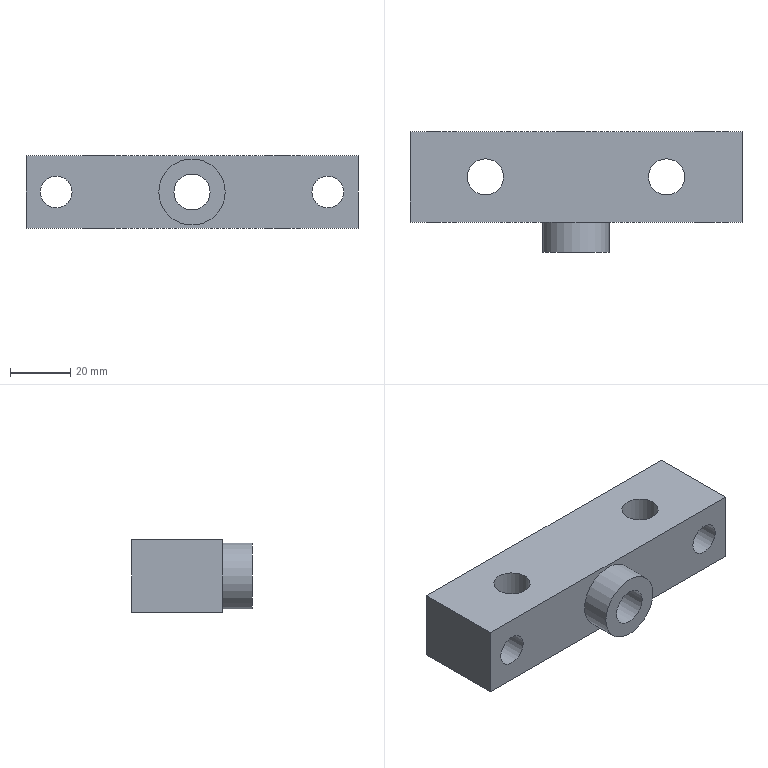Component | NX | MOVING_BLOCK | 1 solid | 13 faces | box 110 x 40 x 24 mm | volume 67853 mm3 | plane 7 | cylinder 6 | commonest cylinder face diameters 12 x3 10.5 x2 22 x1
STEP:
#1=CARTESIAN_POINT('',(0.,0.,0.));
#2=DIRECTION('',(0.,0.,1.));
#3=DIRECTION('',(1.,0.,0.));
#4=AXIS2_PLACEMENT_3D('',#1,#2,#3);
#5=CARTESIAN_POINT('',(85.,-15.,153.));
#6=VERTEX_POINT('',#5);
#7=CARTESIAN_POINT('',(-25.,-15.,153.));
#8=VERTEX_POINT('',#7);
#9=CARTESIAN_POINT('',(85.,-15.,153.));
#10=DIRECTION('',(-1.,0.,0.));
#11=VECTOR('',#10,1.);
#12=LINE('',#9,#11);
#13=CARTESIAN_POINT('',(85.,-15.,129.));
#14=DIRECTION('',(0.,1.,0.));
#15=DIRECTION('',(-1.,0.,0.));
#16=AXIS2_PLACEMENT_3D('',#13,#14,#15);
#17=PLANE('',#16);
#18=CARTESIAN_POINT('',(0.,24.));
#19=DIRECTION('',(1.,0.));
#20=VECTOR('',#19,1.);
#21=LINE('',#18,#20);
#22=(GEOMETRIC_REPRESENTATION_CONTEXT(2)PARAMETRIC_REPRESENTATION_CONTEXT()REPRESENTATION_CONTEXT('',''));
#23=DEFINITIONAL_REPRESENTATION('',(#21),#22);
#24=PCURVE('',#17,#23);
#25=CARTESIAN_POINT('',(-0.,0.,153.));
#26=DIRECTION('',(0.,0.,1.));
#27=DIRECTION('',(0.,-1.,0.));
#28=AXIS2_PLACEMENT_3D('',#25,#26,#27);
#29=PLANE('',#28);
#30=CARTESIAN_POINT('',(15.,85.));
#31=DIRECTION('',(0.,-1.));
#32=VECTOR('',#31,1.);
#33=LINE('',#30,#32);
#34=(GEOMETRIC_REPRESENTATION_CONTEXT(2)PARAMETRIC_REPRESENTATION_CONTEXT()REPRESENTATION_CONTEXT('',''));
#35=DEFINITIONAL_REPRESENTATION('',(#33),#34);
#36=PCURVE('',#29,#35);
#37=SURFACE_CURVE('',#12,(#24,#36),.PCURVE_S1.);
#38=EDGE_CURVE('',#6,#8,#37,.T.);
#39=ORIENTED_EDGE('',*,*,#38,.T.);
#40=CARTESIAN_POINT('',(-25.,-15.,129.));
#41=VERTEX_POINT('',#40);
#42=CARTESIAN_POINT('',(-25.,-15.,129.));
#43=DIRECTION('',(0.,0.,1.));
#44=VECTOR('',#43,1.);
#45=LINE('',#42,#44);
#46=CARTESIAN_POINT('',(110.,0.));
#47=DIRECTION('',(0.,1.));
#48=VECTOR('',#47,1.);
#49=LINE('',#46,#48);
#50=(GEOMETRIC_REPRESENTATION_CONTEXT(2)PARAMETRIC_REPRESENTATION_CONTEXT()REPRESENTATION_CONTEXT('',''));
#51=DEFINITIONAL_REPRESENTATION('',(#49),#50);
#52=PCURVE('',#17,#51);
#53=CARTESIAN_POINT('',(-25.,-15.,129.));
#54=DIRECTION('',(1.,0.,0.));
#55=DIRECTION('',(0.,1.,0.));
#56=AXIS2_PLACEMENT_3D('',#53,#54,#55);
#57=PLANE('',#56);
#58=CARTESIAN_POINT('',(0.,0.));
#59=DIRECTION('',(0.,1.));
#60=VECTOR('',#59,1.);
#61=LINE('',#58,#60);
#62=(GEOMETRIC_REPRESENTATION_CONTEXT(2)PARAMETRIC_REPRESENTATION_CONTEXT()REPRESENTATION_CONTEXT('',''));
#63=DEFINITIONAL_REPRESENTATION('',(#61),#62);
#64=PCURVE('',#57,#63);
#65=SURFACE_CURVE('',#45,(#52,#64),.PCURVE_S1.);
#66=EDGE_CURVE('',#41,#8,#65,.T.);
#67=ORIENTED_EDGE('',*,*,#66,.F.);
#68=CARTESIAN_POINT('',(85.,-15.,129.));
#69=VERTEX_POINT('',#68);
#70=CARTESIAN_POINT('',(85.,-15.,129.));
#71=DIRECTION('',(-1.,0.,0.));
#72=VECTOR('',#71,1.);
#73=LINE('',#70,#72);
#74=CARTESIAN_POINT('',(0.,0.));
#75=DIRECTION('',(1.,0.));
#76=VECTOR('',#75,1.);
#77=LINE('',#74,#76);
#78=(GEOMETRIC_REPRESENTATION_CONTEXT(2)PARAMETRIC_REPRESENTATION_CONTEXT()REPRESENTATION_CONTEXT('',''));
#79=DEFINITIONAL_REPRESENTATION('',(#77),#78);
#80=PCURVE('',#17,#79);
#81=CARTESIAN_POINT('',(-0.,0.,129.));
#82=DIRECTION('',(0.,0.,1.));
#83=DIRECTION('',(0.,-1.,0.));
#84=AXIS2_PLACEMENT_3D('',#81,#82,#83);
#85=PLANE('',#84);
#86=CARTESIAN_POINT('',(15.,85.));
#87=DIRECTION('',(0.,-1.));
#88=VECTOR('',#87,1.);
#89=LINE('',#86,#88);
#90=(GEOMETRIC_REPRESENTATION_CONTEXT(2)PARAMETRIC_REPRESENTATION_CONTEXT()REPRESENTATION_CONTEXT('',''));
#91=DEFINITIONAL_REPRESENTATION('',(#89),#90);
#92=PCURVE('',#85,#91);
#93=SURFACE_CURVE('',#73,(#80,#92),.PCURVE_S1.);
#94=EDGE_CURVE('',#69,#41,#93,.T.);
#95=ORIENTED_EDGE('',*,*,#94,.F.);
#96=CARTESIAN_POINT('',(85.,-15.,129.));
#97=DIRECTION('',(0.,0.,1.));
#98=VECTOR('',#97,1.);
#99=LINE('',#96,#98);
#100=CARTESIAN_POINT('',(0.,0.));
#101=DIRECTION('',(0.,1.));
#102=VECTOR('',#101,1.);
#103=LINE('',#100,#102);
#104=(GEOMETRIC_REPRESENTATION_CONTEXT(2)PARAMETRIC_REPRESENTATION_CONTEXT()REPRESENTATION_CONTEXT('',''));
#105=DEFINITIONAL_REPRESENTATION('',(#103),#104);
#106=PCURVE('',#17,#105);
#107=CARTESIAN_POINT('',(85.,15.,129.));
#108=DIRECTION('',(-1.,0.,0.));
#109=DIRECTION('',(0.,-1.,0.));
#110=AXIS2_PLACEMENT_3D('',#107,#108,#109);
#111=PLANE('',#110);
#112=CARTESIAN_POINT('',(30.,0.));
#113=DIRECTION('',(0.,1.));
#114=VECTOR('',#113,1.);
#115=LINE('',#112,#114);
#116=(GEOMETRIC_REPRESENTATION_CONTEXT(2)PARAMETRIC_REPRESENTATION_CONTEXT()REPRESENTATION_CONTEXT('',''));
#117=DEFINITIONAL_REPRESENTATION('',(#115),#116);
#118=PCURVE('',#111,#117);
#119=SURFACE_CURVE('',#99,(#106,#118),.PCURVE_S1.);
#120=EDGE_CURVE('',#69,#6,#119,.T.);
#121=ORIENTED_EDGE('',*,*,#120,.T.);
#122=EDGE_LOOP('',(#39,#67,#95,#121));
#123=FACE_BOUND('',#122,.T.);
#124=CARTESIAN_POINT('',(-9.75,-15.,141.));
#125=VERTEX_POINT('',#124);
#126=CARTESIAN_POINT('',(-15.,-15.,141.));
#127=DIRECTION('',(0.,-1.,0.));
#128=DIRECTION('',(1.,0.,0.));
#129=AXIS2_PLACEMENT_3D('',#126,#127,#128);
#130=CIRCLE('',#129,5.25);
#131=CARTESIAN_POINT('',(94.75,12.));
#132=CARTESIAN_POINT('',(94.75,21.093));
#133=CARTESIAN_POINT('',(102.625,16.547));
#134=CARTESIAN_POINT('',(110.5,12.));
#135=CARTESIAN_POINT('',(102.625,7.453));
#136=CARTESIAN_POINT('',(94.75,2.907));
#137=CARTESIAN_POINT('',(94.75,12.));
#138=(BOUNDED_CURVE()B_SPLINE_CURVE(2,(#131,#132,#133,#134,#135,#136,#137),.UNSPECIFIED.,.T.,.F.)B_SPLINE_CURVE_WITH_KNOTS((1,2,2,2,2,1),(-2.094,0.,2.094,4.189,6.283,8.378),.UNSPECIFIED.)CURVE()GEOMETRIC_REPRESENTATION_ITEM()RATIONAL_B_SPLINE_CURVE((1.,0.5,1.,0.5,1.,0.5,1.))REPRESENTATION_ITEM(''));
#139=(GEOMETRIC_REPRESENTATION_CONTEXT(2)PARAMETRIC_REPRESENTATION_CONTEXT()REPRESENTATION_CONTEXT('',''));
#140=DEFINITIONAL_REPRESENTATION('',(#138),#139);
#141=PCURVE('',#17,#140);
#142=CARTESIAN_POINT('',(-15.,35.,141.));
#143=DIRECTION('',(0.,-1.,0.));
#144=DIRECTION('',(1.,0.,0.));
#145=AXIS2_PLACEMENT_3D('',#142,#143,#144);
#146=CYLINDRICAL_SURFACE('',#145,5.25);
#147=CARTESIAN_POINT('',(0.,50.));
#148=DIRECTION('',(1.,0.));
#149=VECTOR('',#148,1.);
#150=LINE('',#147,#149);
#151=(GEOMETRIC_REPRESENTATION_CONTEXT(2)PARAMETRIC_REPRESENTATION_CONTEXT()REPRESENTATION_CONTEXT('',''));
#152=DEFINITIONAL_REPRESENTATION('',(#150),#151);
#153=PCURVE('',#146,#152);
#154=SURFACE_CURVE('',#130,(#141,#153),.PCURVE_S1.);
#155=EDGE_CURVE('',#125,#125,#154,.T.);
#156=ORIENTED_EDGE('',*,*,#155,.F.);
#157=EDGE_LOOP('',(#156));
#158=FACE_BOUND('',#157,.T.);
#159=CARTESIAN_POINT('',(69.75,-15.,141.));
#160=VERTEX_POINT('',#159);
#161=CARTESIAN_POINT('',(80.25,-15.,141.));
#162=VERTEX_POINT('',#161);
#163=CARTESIAN_POINT('',(75.,-15.,141.));
#164=DIRECTION('',(0.,1.,0.));
#165=DIRECTION('',(-1.,0.,0.));
#166=AXIS2_PLACEMENT_3D('',#163,#164,#165);
#167=CIRCLE('',#166,5.25);
#168=CARTESIAN_POINT('',(10.,12.));
#169=DIRECTION('',(1.,0.));
#170=AXIS2_PLACEMENT_2D('',#168,#169);
#171=CIRCLE('',#170,5.25);
#172=(GEOMETRIC_REPRESENTATION_CONTEXT(2)PARAMETRIC_REPRESENTATION_CONTEXT()REPRESENTATION_CONTEXT('',''));
#173=DEFINITIONAL_REPRESENTATION('',(#171),#172);
#174=PCURVE('',#17,#173);
#175=CARTESIAN_POINT('',(75.,35.,141.));
#176=DIRECTION('',(0.,-1.,0.));
#177=DIRECTION('',(1.,0.,0.));
#178=AXIS2_PLACEMENT_3D('',#175,#176,#177);
#179=CYLINDRICAL_SURFACE('',#178,5.25);
#180=CARTESIAN_POINT('',(3.142,50.));
#181=DIRECTION('',(-1.,0.));
#182=VECTOR('',#181,1.);
#183=LINE('',#180,#182);
#184=(GEOMETRIC_REPRESENTATION_CONTEXT(2)PARAMETRIC_REPRESENTATION_CONTEXT()REPRESENTATION_CONTEXT('',''));
#185=DEFINITIONAL_REPRESENTATION('',(#183),#184);
#186=PCURVE('',#179,#185);
#187=SURFACE_CURVE('',#167,(#174,#186),.PCURVE_S1.);
#188=EDGE_CURVE('',#160,#162,#187,.T.);
#189=ORIENTED_EDGE('',*,*,#188,.T.);
#190=CARTESIAN_POINT('',(75.,-15.,141.));
#191=DIRECTION('',(0.,1.,0.));
#192=DIRECTION('',(-1.,0.,0.));
#193=AXIS2_PLACEMENT_3D('',#190,#191,#192);
#194=CIRCLE('',#193,5.25);
#195=CARTESIAN_POINT('',(10.,12.));
#196=DIRECTION('',(1.,0.));
#197=AXIS2_PLACEMENT_2D('',#195,#196);
#198=CIRCLE('',#197,5.25);
#199=(GEOMETRIC_REPRESENTATION_CONTEXT(2)PARAMETRIC_REPRESENTATION_CONTEXT()REPRESENTATION_CONTEXT('',''));
#200=DEFINITIONAL_REPRESENTATION('',(#198),#199);
#201=PCURVE('',#17,#200);
#202=CARTESIAN_POINT('',(9.425,50.));
#203=DIRECTION('',(-1.,0.));
#204=VECTOR('',#203,1.);
#205=LINE('',#202,#204);
#206=(GEOMETRIC_REPRESENTATION_CONTEXT(2)PARAMETRIC_REPRESENTATION_CONTEXT()REPRESENTATION_CONTEXT('',''));
#207=DEFINITIONAL_REPRESENTATION('',(#205),#206);
#208=PCURVE('',#179,#207);
#209=SURFACE_CURVE('',#194,(#201,#208),.PCURVE_S1.);
#210=EDGE_CURVE('',#162,#160,#209,.T.);
#211=ORIENTED_EDGE('',*,*,#210,.T.);
#212=EDGE_LOOP('',(#189,#211));
#213=FACE_BOUND('',#212,.T.);
#214=CARTESIAN_POINT('',(41.,-15.,141.));
#215=VERTEX_POINT('',#214);
#216=CARTESIAN_POINT('',(30.,-15.,141.));
#217=DIRECTION('',(0.,-1.,0.));
#218=DIRECTION('',(1.,0.,0.));
#219=AXIS2_PLACEMENT_3D('',#216,#217,#218);
#220=CIRCLE('',#219,11.);
#221=CARTESIAN_POINT('',(44.,12.));
#222=CARTESIAN_POINT('',(44.,31.053));
#223=CARTESIAN_POINT('',(60.5,21.526));
#224=CARTESIAN_POINT('',(77.,12.));
#225=CARTESIAN_POINT('',(60.5,2.474));
#226=CARTESIAN_POINT('',(44.,-7.053));
#227=CARTESIAN_POINT('',(44.,12.));
#228=(BOUNDED_CURVE()B_SPLINE_CURVE(2,(#221,#222,#223,#224,#225,#226,#227),.UNSPECIFIED.,.T.,.F.)B_SPLINE_CURVE_WITH_KNOTS((1,2,2,2,2,1),(-2.094,0.,2.094,4.189,6.283,8.378),.UNSPECIFIED.)CURVE()GEOMETRIC_REPRESENTATION_ITEM()RATIONAL_B_SPLINE_CURVE((1.,0.5,1.,0.5,1.,0.5,1.))REPRESENTATION_ITEM(''));
#229=(GEOMETRIC_REPRESENTATION_CONTEXT(2)PARAMETRIC_REPRESENTATION_CONTEXT()REPRESENTATION_CONTEXT('',''));
#230=DEFINITIONAL_REPRESENTATION('',(#228),#229);
#231=PCURVE('',#17,#230);
#232=CARTESIAN_POINT('',(30.,-25.,141.));
#233=DIRECTION('',(0.,1.,0.));
#234=DIRECTION('',(-1.,0.,0.));
#235=AXIS2_PLACEMENT_3D('',#232,#233,#234);
#236=CYLINDRICAL_SURFACE('',#235,11.);
#237=CARTESIAN_POINT('',(9.425,10.));
#238=DIRECTION('',(-1.,0.));
#239=VECTOR('',#238,1.);
#240=LINE('',#237,#239);
#241=(GEOMETRIC_REPRESENTATION_CONTEXT(2)PARAMETRIC_REPRESENTATION_CONTEXT()REPRESENTATION_CONTEXT('',''));
#242=DEFINITIONAL_REPRESENTATION('',(#240),#241);
#243=PCURVE('',#236,#242);
#244=SURFACE_CURVE('',#220,(#231,#243),.PCURVE_S1.);
#245=EDGE_CURVE('',#215,#215,#244,.T.);
#246=ORIENTED_EDGE('',*,*,#245,.F.);
#247=EDGE_LOOP('',(#246));
#248=FACE_BOUND('',#247,.T.);
#249=ADVANCED_FACE('',(#123,#158,#213,#248),#17,.F.);
#250=CARTESIAN_POINT('',(-25.,15.,153.));
#251=VERTEX_POINT('',#250);
#252=CARTESIAN_POINT('',(-25.,-15.,153.));
#253=DIRECTION('',(0.,1.,0.));
#254=VECTOR('',#253,1.);
#255=LINE('',#252,#254);
#256=CARTESIAN_POINT('',(0.,24.));
#257=DIRECTION('',(1.,0.));
#258=VECTOR('',#257,1.);
#259=LINE('',#256,#258);
#260=(GEOMETRIC_REPRESENTATION_CONTEXT(2)PARAMETRIC_REPRESENTATION_CONTEXT()REPRESENTATION_CONTEXT('',''));
#261=DEFINITIONAL_REPRESENTATION('',(#259),#260);
#262=PCURVE('',#57,#261);
#263=CARTESIAN_POINT('',(15.,-25.));
#264=DIRECTION('',(-1.,0.));
#265=VECTOR('',#264,1.);
#266=LINE('',#263,#265);
#267=(GEOMETRIC_REPRESENTATION_CONTEXT(2)PARAMETRIC_REPRESENTATION_CONTEXT()REPRESENTATION_CONTEXT('',''));
#268=DEFINITIONAL_REPRESENTATION('',(#266),#267);
#269=PCURVE('',#29,#268);
#270=SURFACE_CURVE('',#255,(#262,#269),.PCURVE_S1.);
#271=EDGE_CURVE('',#8,#251,#270,.T.);
#272=ORIENTED_EDGE('',*,*,#271,.T.);
#273=CARTESIAN_POINT('',(-25.,15.,129.));
#274=VERTEX_POINT('',#273);
#275=CARTESIAN_POINT('',(-25.,15.,129.));
#276=DIRECTION('',(0.,0.,1.));
#277=VECTOR('',#276,1.);
#278=LINE('',#275,#277);
#279=CARTESIAN_POINT('',(30.,0.));
#280=DIRECTION('',(0.,1.));
#281=VECTOR('',#280,1.);
#282=LINE('',#279,#281);
#283=(GEOMETRIC_REPRESENTATION_CONTEXT(2)PARAMETRIC_REPRESENTATION_CONTEXT()REPRESENTATION_CONTEXT('',''));
#284=DEFINITIONAL_REPRESENTATION('',(#282),#283);
#285=PCURVE('',#57,#284);
#286=CARTESIAN_POINT('',(-25.,15.,129.));
#287=DIRECTION('',(0.,-1.,0.));
#288=DIRECTION('',(1.,0.,0.));
#289=AXIS2_PLACEMENT_3D('',#286,#287,#288);
#290=PLANE('',#289);
#291=CARTESIAN_POINT('',(0.,0.));
#292=DIRECTION('',(0.,1.));
#293=VECTOR('',#292,1.);
#294=LINE('',#291,#293);
#295=(GEOMETRIC_REPRESENTATION_CONTEXT(2)PARAMETRIC_REPRESENTATION_CONTEXT()REPRESENTATION_CONTEXT('',''));
#296=DEFINITIONAL_REPRESENTATION('',(#294),#295);
#297=PCURVE('',#290,#296);
#298=SURFACE_CURVE('',#278,(#285,#297),.PCURVE_S1.);
#299=EDGE_CURVE('',#274,#251,#298,.T.);
#300=ORIENTED_EDGE('',*,*,#299,.F.);
#301=CARTESIAN_POINT('',(-25.,-15.,129.));
#302=DIRECTION('',(0.,1.,0.));
#303=VECTOR('',#302,1.);
#304=LINE('',#301,#303);
#305=CARTESIAN_POINT('',(0.,0.));
#306=DIRECTION('',(1.,0.));
#307=VECTOR('',#306,1.);
#308=LINE('',#305,#307);
#309=(GEOMETRIC_REPRESENTATION_CONTEXT(2)PARAMETRIC_REPRESENTATION_CONTEXT()REPRESENTATION_CONTEXT('',''));
#310=DEFINITIONAL_REPRESENTATION('',(#308),#309);
#311=PCURVE('',#57,#310);
#312=CARTESIAN_POINT('',(15.,-25.));
#313=DIRECTION('',(-1.,0.));
#314=VECTOR('',#313,1.);
#315=LINE('',#312,#314);
#316=(GEOMETRIC_REPRESENTATION_CONTEXT(2)PARAMETRIC_REPRESENTATION_CONTEXT()REPRESENTATION_CONTEXT('',''));
#317=DEFINITIONAL_REPRESENTATION('',(#315),#316);
#318=PCURVE('',#85,#317);
#319=SURFACE_CURVE('',#304,(#311,#318),.PCURVE_S1.);
#320=EDGE_CURVE('',#41,#274,#319,.T.);
#321=ORIENTED_EDGE('',*,*,#320,.F.);
#322=ORIENTED_EDGE('',*,*,#66,.T.);
#323=EDGE_LOOP('',(#272,#300,#321,#322));
#324=FACE_BOUND('',#323,.T.);
#325=ADVANCED_FACE('',(#324),#57,.F.);
#326=CARTESIAN_POINT('',(80.25,15.,141.));
#327=VERTEX_POINT('',#326);
#328=CARTESIAN_POINT('',(75.,15.,141.));
#329=DIRECTION('',(0.,1.,0.));
#330=DIRECTION('',(1.,0.,0.));
#331=AXIS2_PLACEMENT_3D('',#328,#329,#330);
#332=CIRCLE('',#331,5.25);
#333=CARTESIAN_POINT('',(105.25,12.));
#334=CARTESIAN_POINT('',(105.25,2.907));
#335=CARTESIAN_POINT('',(97.375,7.453));
#336=CARTESIAN_POINT('',(89.5,12.));
#337=CARTESIAN_POINT('',(97.375,16.547));
#338=CARTESIAN_POINT('',(105.25,21.093));
#339=CARTESIAN_POINT('',(105.25,12.));
#340=(BOUNDED_CURVE()B_SPLINE_CURVE(2,(#333,#334,#335,#336,#337,#338,#339),.UNSPECIFIED.,.T.,.F.)B_SPLINE_CURVE_WITH_KNOTS((1,2,2,2,2,1),(-2.094,0.,2.094,4.189,6.283,8.378),.UNSPECIFIED.)CURVE()GEOMETRIC_REPRESENTATION_ITEM()RATIONAL_B_SPLINE_CURVE((1.,0.5,1.,0.5,1.,0.5,1.))REPRESENTATION_ITEM(''));
#341=(GEOMETRIC_REPRESENTATION_CONTEXT(2)PARAMETRIC_REPRESENTATION_CONTEXT()REPRESENTATION_CONTEXT('',''));
#342=DEFINITIONAL_REPRESENTATION('',(#340),#341);
#343=PCURVE('',#290,#342);
#344=CARTESIAN_POINT('',(6.283,20.));
#345=DIRECTION('',(-1.,0.));
#346=VECTOR('',#345,1.);
#347=LINE('',#344,#346);
#348=(GEOMETRIC_REPRESENTATION_CONTEXT(2)PARAMETRIC_REPRESENTATION_CONTEXT()REPRESENTATION_CONTEXT('',''));
#349=DEFINITIONAL_REPRESENTATION('',(#347),#348);
#350=PCURVE('',#179,#349);
#351=SURFACE_CURVE('',#332,(#343,#350),.PCURVE_S1.);
#352=EDGE_CURVE('',#327,#327,#351,.T.);
#353=ORIENTED_EDGE('',*,*,#352,.F.);
#354=EDGE_LOOP('',(#353));
#355=FACE_BOUND('',#354,.T.);
#356=CARTESIAN_POINT('',(-9.75,15.,141.));
#357=VERTEX_POINT('',#356);
#358=CARTESIAN_POINT('',(-15.,15.,141.));
#359=DIRECTION('',(0.,-1.,0.));
#360=DIRECTION('',(1.,0.,0.));
#361=AXIS2_PLACEMENT_3D('',#358,#359,#360);
#362=CIRCLE('',#361,5.25);
#363=CARTESIAN_POINT('',(10.,12.));
#364=DIRECTION('',(1.,0.));
#365=AXIS2_PLACEMENT_2D('',#363,#364);
#366=CIRCLE('',#365,5.25);
#367=(GEOMETRIC_REPRESENTATION_CONTEXT(2)PARAMETRIC_REPRESENTATION_CONTEXT()REPRESENTATION_CONTEXT('',''));
#368=DEFINITIONAL_REPRESENTATION('',(#366),#367);
#369=PCURVE('',#290,#368);
#370=CARTESIAN_POINT('',(0.,20.));
#371=DIRECTION('',(1.,0.));
#372=VECTOR('',#371,1.);
#373=LINE('',#370,#372);
#374=(GEOMETRIC_REPRESENTATION_CONTEXT(2)PARAMETRIC_REPRESENTATION_CONTEXT()REPRESENTATION_CONTEXT('',''));
#375=DEFINITIONAL_REPRESENTATION('',(#373),#374);
#376=PCURVE('',#146,#375);
#377=SURFACE_CURVE('',#362,(#369,#376),.PCURVE_S1.);
#378=EDGE_CURVE('',#357,#357,#377,.T.);
#379=ORIENTED_EDGE('',*,*,#378,.T.);
#380=EDGE_LOOP('',(#379));
#381=FACE_BOUND('',#380,.T.);
#382=CARTESIAN_POINT('',(36.,15.,141.));
#383=VERTEX_POINT('',#382);
#384=CARTESIAN_POINT('',(30.,15.,141.));
#385=DIRECTION('',(0.,1.,0.));
#386=DIRECTION('',(1.,0.,0.));
#387=AXIS2_PLACEMENT_3D('',#384,#385,#386);
#388=CIRCLE('',#387,6.);
#389=CARTESIAN_POINT('',(61.,12.));
#390=CARTESIAN_POINT('',(61.,1.608));
#391=CARTESIAN_POINT('',(52.,6.804));
#392=CARTESIAN_POINT('',(43.,12.));
#393=CARTESIAN_POINT('',(52.,17.196));
#394=CARTESIAN_POINT('',(61.,22.392));
#395=CARTESIAN_POINT('',(61.,12.));
#396=(BOUNDED_CURVE()B_SPLINE_CURVE(2,(#389,#390,#391,#392,#393,#394,#395),.UNSPECIFIED.,.T.,.F.)B_SPLINE_CURVE_WITH_KNOTS((1,2,2,2,2,1),(-2.094,0.,2.094,4.189,6.283,8.378),.UNSPECIFIED.)CURVE()GEOMETRIC_REPRESENTATION_ITEM()RATIONAL_B_SPLINE_CURVE((1.,0.5,1.,0.5,1.,0.5,1.))REPRESENTATION_ITEM(''));
#397=(GEOMETRIC_REPRESENTATION_CONTEXT(2)PARAMETRIC_REPRESENTATION_CONTEXT()REPRESENTATION_CONTEXT('',''));
#398=DEFINITIONAL_REPRESENTATION('',(#396),#397);
#399=PCURVE('',#290,#398);
#400=CARTESIAN_POINT('',(30.,35.,141.));
#401=DIRECTION('',(0.,-1.,0.));
#402=DIRECTION('',(1.,0.,0.));
#403=AXIS2_PLACEMENT_3D('',#400,#401,#402);
#404=CYLINDRICAL_SURFACE('',#403,6.);
#405=CARTESIAN_POINT('',(6.283,20.));
#406=DIRECTION('',(-1.,0.));
#407=VECTOR('',#406,1.);
#408=LINE('',#405,#407);
#409=(GEOMETRIC_REPRESENTATION_CONTEXT(2)PARAMETRIC_REPRESENTATION_CONTEXT()REPRESENTATION_CONTEXT('',''));
#410=DEFINITIONAL_REPRESENTATION('',(#408),#409);
#411=PCURVE('',#404,#410);
#412=SURFACE_CURVE('',#388,(#399,#411),.PCURVE_S1.);
#413=EDGE_CURVE('',#383,#383,#412,.T.);
#414=ORIENTED_EDGE('',*,*,#413,.F.);
#415=EDGE_LOOP('',(#414));
#416=FACE_BOUND('',#415,.T.);
#417=CARTESIAN_POINT('',(85.,15.,153.));
#418=VERTEX_POINT('',#417);
#419=CARTESIAN_POINT('',(-25.,15.,153.));
#420=DIRECTION('',(1.,0.,0.));
#421=VECTOR('',#420,1.);
#422=LINE('',#419,#421);
#423=CARTESIAN_POINT('',(0.,24.));
#424=DIRECTION('',(1.,0.));
#425=VECTOR('',#424,1.);
#426=LINE('',#423,#425);
#427=(GEOMETRIC_REPRESENTATION_CONTEXT(2)PARAMETRIC_REPRESENTATION_CONTEXT()REPRESENTATION_CONTEXT('',''));
#428=DEFINITIONAL_REPRESENTATION('',(#426),#427);
#429=PCURVE('',#290,#428);
#430=CARTESIAN_POINT('',(-15.,-25.));
#431=DIRECTION('',(0.,1.));
#432=VECTOR('',#431,1.);
#433=LINE('',#430,#432);
#434=(GEOMETRIC_REPRESENTATION_CONTEXT(2)PARAMETRIC_REPRESENTATION_CONTEXT()REPRESENTATION_CONTEXT('',''));
#435=DEFINITIONAL_REPRESENTATION('',(#433),#434);
#436=PCURVE('',#29,#435);
#437=SURFACE_CURVE('',#422,(#429,#436),.PCURVE_S1.);
#438=EDGE_CURVE('',#251,#418,#437,.T.);
#439=ORIENTED_EDGE('',*,*,#438,.T.);
#440=CARTESIAN_POINT('',(85.,15.,129.));
#441=VERTEX_POINT('',#440);
#442=CARTESIAN_POINT('',(85.,15.,129.));
#443=DIRECTION('',(0.,0.,1.));
#444=VECTOR('',#443,1.);
#445=LINE('',#442,#444);
#446=CARTESIAN_POINT('',(110.,0.));
#447=DIRECTION('',(0.,1.));
#448=VECTOR('',#447,1.);
#449=LINE('',#446,#448);
#450=(GEOMETRIC_REPRESENTATION_CONTEXT(2)PARAMETRIC_REPRESENTATION_CONTEXT()REPRESENTATION_CONTEXT('',''));
#451=DEFINITIONAL_REPRESENTATION('',(#449),#450);
#452=PCURVE('',#290,#451);
#453=CARTESIAN_POINT('',(0.,0.));
#454=DIRECTION('',(0.,1.));
#455=VECTOR('',#454,1.);
#456=LINE('',#453,#455);
#457=(GEOMETRIC_REPRESENTATION_CONTEXT(2)PARAMETRIC_REPRESENTATION_CONTEXT()REPRESENTATION_CONTEXT('',''));
#458=DEFINITIONAL_REPRESENTATION('',(#456),#457);
#459=PCURVE('',#111,#458);
#460=SURFACE_CURVE('',#445,(#452,#459),.PCURVE_S1.);
#461=EDGE_CURVE('',#441,#418,#460,.T.);
#462=ORIENTED_EDGE('',*,*,#461,.F.);
#463=CARTESIAN_POINT('',(-25.,15.,129.));
#464=DIRECTION('',(1.,0.,0.));
#465=VECTOR('',#464,1.);
#466=LINE('',#463,#465);
#467=CARTESIAN_POINT('',(0.,0.));
#468=DIRECTION('',(1.,0.));
#469=VECTOR('',#468,1.);
#470=LINE('',#467,#469);
#471=(GEOMETRIC_REPRESENTATION_CONTEXT(2)PARAMETRIC_REPRESENTATION_CONTEXT()REPRESENTATION_CONTEXT('',''));
#472=DEFINITIONAL_REPRESENTATION('',(#470),#471);
#473=PCURVE('',#290,#472);
#474=CARTESIAN_POINT('',(-15.,-25.));
#475=DIRECTION('',(0.,1.));
#476=VECTOR('',#475,1.);
#477=LINE('',#474,#476);
#478=(GEOMETRIC_REPRESENTATION_CONTEXT(2)PARAMETRIC_REPRESENTATION_CONTEXT()REPRESENTATION_CONTEXT('',''));
#479=DEFINITIONAL_REPRESENTATION('',(#477),#478);
#480=PCURVE('',#85,#479);
#481=SURFACE_CURVE('',#466,(#473,#480),.PCURVE_S1.);
#482=EDGE_CURVE('',#274,#441,#481,.T.);
#483=ORIENTED_EDGE('',*,*,#482,.F.);
#484=ORIENTED_EDGE('',*,*,#299,.T.);
#485=EDGE_LOOP('',(#439,#462,#483,#484));
#486=FACE_BOUND('',#485,.T.);
#487=ADVANCED_FACE('',(#355,#381,#416,#486),#290,.F.);
#488=CARTESIAN_POINT('',(85.,15.,153.));
#489=DIRECTION('',(0.,-1.,0.));
#490=VECTOR('',#489,1.);
#491=LINE('',#488,#490);
#492=CARTESIAN_POINT('',(0.,24.));
#493=DIRECTION('',(1.,0.));
#494=VECTOR('',#493,1.);
#495=LINE('',#492,#494);
#496=(GEOMETRIC_REPRESENTATION_CONTEXT(2)PARAMETRIC_REPRESENTATION_CONTEXT()REPRESENTATION_CONTEXT('',''));
#497=DEFINITIONAL_REPRESENTATION('',(#495),#496);
#498=PCURVE('',#111,#497);
#499=CARTESIAN_POINT('',(-15.,85.));
#500=DIRECTION('',(1.,0.));
#501=VECTOR('',#500,1.);
#502=LINE('',#499,#501);
#503=(GEOMETRIC_REPRESENTATION_CONTEXT(2)PARAMETRIC_REPRESENTATION_CONTEXT()REPRESENTATION_CONTEXT('',''));
#504=DEFINITIONAL_REPRESENTATION('',(#502),#503);
#505=PCURVE('',#29,#504);
#506=SURFACE_CURVE('',#491,(#498,#505),.PCURVE_S1.);
#507=EDGE_CURVE('',#418,#6,#506,.T.);
#508=ORIENTED_EDGE('',*,*,#507,.T.);
#509=ORIENTED_EDGE('',*,*,#120,.F.);
#510=CARTESIAN_POINT('',(85.,15.,129.));
#511=DIRECTION('',(0.,-1.,0.));
#512=VECTOR('',#511,1.);
#513=LINE('',#510,#512);
#514=CARTESIAN_POINT('',(0.,0.));
#515=DIRECTION('',(1.,0.));
#516=VECTOR('',#515,1.);
#517=LINE('',#514,#516);
#518=(GEOMETRIC_REPRESENTATION_CONTEXT(2)PARAMETRIC_REPRESENTATION_CONTEXT()REPRESENTATION_CONTEXT('',''));
#519=DEFINITIONAL_REPRESENTATION('',(#517),#518);
#520=PCURVE('',#111,#519);
#521=CARTESIAN_POINT('',(-15.,85.));
#522=DIRECTION('',(1.,0.));
#523=VECTOR('',#522,1.);
#524=LINE('',#521,#523);
#525=(GEOMETRIC_REPRESENTATION_CONTEXT(2)PARAMETRIC_REPRESENTATION_CONTEXT()REPRESENTATION_CONTEXT('',''));
#526=DEFINITIONAL_REPRESENTATION('',(#524),#525);
#527=PCURVE('',#85,#526);
#528=SURFACE_CURVE('',#513,(#520,#527),.PCURVE_S1.);
#529=EDGE_CURVE('',#441,#69,#528,.T.);
#530=ORIENTED_EDGE('',*,*,#529,.F.);
#531=ORIENTED_EDGE('',*,*,#461,.T.);
#532=EDGE_LOOP('',(#508,#509,#530,#531));
#533=FACE_BOUND('',#532,.T.);
#534=ADVANCED_FACE('',(#533),#111,.F.);
#535=CARTESIAN_POINT('',(-0.,-6.,129.));
#536=VERTEX_POINT('',#535);
#537=CARTESIAN_POINT('',(-0.,0.,129.));
#538=DIRECTION('',(0.,0.,1.));
#539=DIRECTION('',(0.,-1.,0.));
#540=AXIS2_PLACEMENT_3D('',#537,#538,#539);
#541=CIRCLE('',#540,6.);
#542=CARTESIAN_POINT('',(-0.,0.,129.));
#543=DIRECTION('',(0.,0.,1.));
#544=DIRECTION('',(0.,-1.,0.));
#545=AXIS2_PLACEMENT_3D('',#542,#543,#544);
#546=CYLINDRICAL_SURFACE('',#545,6.);
#547=CARTESIAN_POINT('',(0.,0.));
#548=DIRECTION('',(1.,0.));
#549=VECTOR('',#548,1.);
#550=LINE('',#547,#549);
#551=(GEOMETRIC_REPRESENTATION_CONTEXT(2)PARAMETRIC_REPRESENTATION_CONTEXT()REPRESENTATION_CONTEXT('',''));
#552=DEFINITIONAL_REPRESENTATION('',(#550),#551);
#553=PCURVE('',#546,#552);
#554=CARTESIAN_POINT('',(0.,0.));
#555=DIRECTION('',(1.,0.));
#556=AXIS2_PLACEMENT_2D('',#554,#555);
#557=CIRCLE('',#556,6.);
#558=(GEOMETRIC_REPRESENTATION_CONTEXT(2)PARAMETRIC_REPRESENTATION_CONTEXT()REPRESENTATION_CONTEXT('',''));
#559=DEFINITIONAL_REPRESENTATION('',(#557),#558);
#560=PCURVE('',#85,#559);
#561=SURFACE_CURVE('',#541,(#553,#560),.PCURVE_S1.);
#562=EDGE_CURVE('',#536,#536,#561,.T.);
#563=ORIENTED_EDGE('',*,*,#562,.T.);
#564=CARTESIAN_POINT('',(-0.,-6.,153.));
#565=VERTEX_POINT('',#564);
#566=CARTESIAN_POINT('',(-0.,-6.,129.));
#567=CARTESIAN_POINT('',(-0.,-6.,153.));
#568=B_SPLINE_CURVE_WITH_KNOTS('',1,(#566,#567),.UNSPECIFIED.,.F.,.F.,(2,2),(0.,24.),.PIECEWISE_BEZIER_KNOTS.);
#569=CARTESIAN_POINT('',(6.283,0.));
#570=DIRECTION('',(0.,1.));
#571=VECTOR('',#570,1.);
#572=LINE('',#569,#571);
#573=(GEOMETRIC_REPRESENTATION_CONTEXT(2)PARAMETRIC_REPRESENTATION_CONTEXT()REPRESENTATION_CONTEXT('',''));
#574=DEFINITIONAL_REPRESENTATION('',(#572),#573);
#575=PCURVE('',#546,#574);
#576=CARTESIAN_POINT('',(0.,0.));
#577=DIRECTION('',(0.,1.));
#578=VECTOR('',#577,1.);
#579=LINE('',#576,#578);
#580=(GEOMETRIC_REPRESENTATION_CONTEXT(2)PARAMETRIC_REPRESENTATION_CONTEXT()REPRESENTATION_CONTEXT('',''));
#581=DEFINITIONAL_REPRESENTATION('',(#579),#580);
#582=PCURVE('',#546,#581);
#583=SEAM_CURVE('',#568,(#575,#582),.PCURVE_S1.);
#584=EDGE_CURVE('',#536,#565,#583,.T.);
#585=ORIENTED_EDGE('',*,*,#584,.T.);
#586=CARTESIAN_POINT('',(-0.,0.,153.));
#587=DIRECTION('',(0.,0.,1.));
#588=DIRECTION('',(0.,-1.,0.));
#589=AXIS2_PLACEMENT_3D('',#586,#587,#588);
#590=CIRCLE('',#589,6.);
#591=CARTESIAN_POINT('',(0.,24.));
#592=DIRECTION('',(1.,0.));
#593=VECTOR('',#592,1.);
#594=LINE('',#591,#593);
#595=(GEOMETRIC_REPRESENTATION_CONTEXT(2)PARAMETRIC_REPRESENTATION_CONTEXT()REPRESENTATION_CONTEXT('',''));
#596=DEFINITIONAL_REPRESENTATION('',(#594),#595);
#597=PCURVE('',#546,#596);
#598=CARTESIAN_POINT('',(0.,0.));
#599=DIRECTION('',(1.,0.));
#600=AXIS2_PLACEMENT_2D('',#598,#599);
#601=CIRCLE('',#600,6.);
#602=(GEOMETRIC_REPRESENTATION_CONTEXT(2)PARAMETRIC_REPRESENTATION_CONTEXT()REPRESENTATION_CONTEXT('',''));
#603=DEFINITIONAL_REPRESENTATION('',(#601),#602);
#604=PCURVE('',#29,#603);
#605=SURFACE_CURVE('',#590,(#597,#604),.PCURVE_S1.);
#606=EDGE_CURVE('',#565,#565,#605,.T.);
#607=ORIENTED_EDGE('',*,*,#606,.F.);
#608=ORIENTED_EDGE('',*,*,#584,.F.);
#609=EDGE_LOOP('',(#563,#585,#607,#608));
#610=FACE_BOUND('',#609,.F.);
#611=ADVANCED_FACE('',(#610),#546,.F.);
#612=CARTESIAN_POINT('',(60.,-6.,129.));
#613=VERTEX_POINT('',#612);
#614=CARTESIAN_POINT('',(60.,0.,129.));
#615=DIRECTION('',(0.,0.,-1.));
#616=DIRECTION('',(0.,-1.,0.));
#617=AXIS2_PLACEMENT_3D('',#614,#615,#616);
#618=CIRCLE('',#617,6.);
#619=CARTESIAN_POINT('',(60.,0.,129.));
#620=DIRECTION('',(0.,0.,1.));
#621=DIRECTION('',(0.,-1.,0.));
#622=AXIS2_PLACEMENT_3D('',#619,#620,#621);
#623=CYLINDRICAL_SURFACE('',#622,6.);
#624=CARTESIAN_POINT('',(6.283,0.));
#625=DIRECTION('',(-1.,0.));
#626=VECTOR('',#625,1.);
#627=LINE('',#624,#626);
#628=(GEOMETRIC_REPRESENTATION_CONTEXT(2)PARAMETRIC_REPRESENTATION_CONTEXT()REPRESENTATION_CONTEXT('',''));
#629=DEFINITIONAL_REPRESENTATION('',(#627),#628);
#630=PCURVE('',#623,#629);
#631=CARTESIAN_POINT('',(6.,60.));
#632=CARTESIAN_POINT('',(6.,49.608));
#633=CARTESIAN_POINT('',(-3.,54.804));
#634=CARTESIAN_POINT('',(-12.,60.));
#635=CARTESIAN_POINT('',(-3.,65.196));
#636=CARTESIAN_POINT('',(6.,70.392));
#637=CARTESIAN_POINT('',(6.,60.));
#638=(BOUNDED_CURVE()B_SPLINE_CURVE(2,(#631,#632,#633,#634,#635,#636,#637),.UNSPECIFIED.,.T.,.F.)B_SPLINE_CURVE_WITH_KNOTS((1,2,2,2,2,1),(-2.094,0.,2.094,4.189,6.283,8.378),.UNSPECIFIED.)CURVE()GEOMETRIC_REPRESENTATION_ITEM()RATIONAL_B_SPLINE_CURVE((1.,0.5,1.,0.5,1.,0.5,1.))REPRESENTATION_ITEM(''));
#639=(GEOMETRIC_REPRESENTATION_CONTEXT(2)PARAMETRIC_REPRESENTATION_CONTEXT()REPRESENTATION_CONTEXT('',''));
#640=DEFINITIONAL_REPRESENTATION('',(#638),#639);
#641=PCURVE('',#85,#640);
#642=SURFACE_CURVE('',#618,(#630,#641),.PCURVE_S1.);
#643=EDGE_CURVE('',#613,#613,#642,.T.);
#644=ORIENTED_EDGE('',*,*,#643,.F.);
#645=CARTESIAN_POINT('',(60.,-6.,153.));
#646=VERTEX_POINT('',#645);
#647=CARTESIAN_POINT('',(60.,-6.,129.));
#648=CARTESIAN_POINT('',(60.,-6.,153.));
#649=B_SPLINE_CURVE_WITH_KNOTS('',1,(#647,#648),.UNSPECIFIED.,.F.,.F.,(2,2),(0.,24.),.PIECEWISE_BEZIER_KNOTS.);
#650=CARTESIAN_POINT('',(6.283,0.));
#651=DIRECTION('',(0.,1.));
#652=VECTOR('',#651,1.);
#653=LINE('',#650,#652);
#654=(GEOMETRIC_REPRESENTATION_CONTEXT(2)PARAMETRIC_REPRESENTATION_CONTEXT()REPRESENTATION_CONTEXT('',''));
#655=DEFINITIONAL_REPRESENTATION('',(#653),#654);
#656=PCURVE('',#623,#655);
#657=CARTESIAN_POINT('',(0.,0.));
#658=DIRECTION('',(0.,1.));
#659=VECTOR('',#658,1.);
#660=LINE('',#657,#659);
#661=(GEOMETRIC_REPRESENTATION_CONTEXT(2)PARAMETRIC_REPRESENTATION_CONTEXT()REPRESENTATION_CONTEXT('',''));
#662=DEFINITIONAL_REPRESENTATION('',(#660),#661);
#663=PCURVE('',#623,#662);
#664=SEAM_CURVE('',#649,(#656,#663),.PCURVE_S1.);
#665=EDGE_CURVE('',#613,#646,#664,.T.);
#666=ORIENTED_EDGE('',*,*,#665,.T.);
#667=CARTESIAN_POINT('',(60.,0.,153.));
#668=DIRECTION('',(0.,0.,-1.));
#669=DIRECTION('',(0.,-1.,0.));
#670=AXIS2_PLACEMENT_3D('',#667,#668,#669);
#671=CIRCLE('',#670,6.);
#672=CARTESIAN_POINT('',(6.283,24.));
#673=DIRECTION('',(-1.,0.));
#674=VECTOR('',#673,1.);
#675=LINE('',#672,#674);
#676=(GEOMETRIC_REPRESENTATION_CONTEXT(2)PARAMETRIC_REPRESENTATION_CONTEXT()REPRESENTATION_CONTEXT('',''));
#677=DEFINITIONAL_REPRESENTATION('',(#675),#676);
#678=PCURVE('',#623,#677);
#679=CARTESIAN_POINT('',(6.,60.));
#680=CARTESIAN_POINT('',(6.,49.608));
#681=CARTESIAN_POINT('',(-3.,54.804));
#682=CARTESIAN_POINT('',(-12.,60.));
#683=CARTESIAN_POINT('',(-3.,65.196));
#684=CARTESIAN_POINT('',(6.,70.392));
#685=CARTESIAN_POINT('',(6.,60.));
#686=(BOUNDED_CURVE()B_SPLINE_CURVE(2,(#679,#680,#681,#682,#683,#684,#685),.UNSPECIFIED.,.T.,.F.)B_SPLINE_CURVE_WITH_KNOTS((1,2,2,2,2,1),(-2.094,0.,2.094,4.189,6.283,8.378),.UNSPECIFIED.)CURVE()GEOMETRIC_REPRESENTATION_ITEM()RATIONAL_B_SPLINE_CURVE((1.,0.5,1.,0.5,1.,0.5,1.))REPRESENTATION_ITEM(''));
#687=(GEOMETRIC_REPRESENTATION_CONTEXT(2)PARAMETRIC_REPRESENTATION_CONTEXT()REPRESENTATION_CONTEXT('',''));
#688=DEFINITIONAL_REPRESENTATION('',(#686),#687);
#689=PCURVE('',#29,#688);
#690=SURFACE_CURVE('',#671,(#678,#689),.PCURVE_S1.);
#691=EDGE_CURVE('',#646,#646,#690,.T.);
#692=ORIENTED_EDGE('',*,*,#691,.T.);
#693=ORIENTED_EDGE('',*,*,#665,.F.);
#694=EDGE_LOOP('',(#644,#666,#692,#693));
#695=FACE_BOUND('',#694,.F.);
#696=ADVANCED_FACE('',(#695),#623,.F.);
#697=ORIENTED_EDGE('',*,*,#320,.T.);
#698=ORIENTED_EDGE('',*,*,#482,.T.);
#699=ORIENTED_EDGE('',*,*,#529,.T.);
#700=ORIENTED_EDGE('',*,*,#94,.T.);
#701=EDGE_LOOP('',(#697,#698,#699,#700));
#702=FACE_BOUND('',#701,.T.);
#703=ORIENTED_EDGE('',*,*,#562,.T.);
#704=EDGE_LOOP('',(#703));
#705=FACE_BOUND('',#704,.T.);
#706=ORIENTED_EDGE('',*,*,#643,.F.);
#707=EDGE_LOOP('',(#706));
#708=FACE_BOUND('',#707,.T.);
#709=ADVANCED_FACE('',(#702,#705,#708),#85,.F.);
#710=ORIENTED_EDGE('',*,*,#271,.F.);
#711=ORIENTED_EDGE('',*,*,#38,.F.);
#712=ORIENTED_EDGE('',*,*,#507,.F.);
#713=ORIENTED_EDGE('',*,*,#438,.F.);
#714=EDGE_LOOP('',(#710,#711,#712,#713));
#715=FACE_BOUND('',#714,.T.);
#716=ORIENTED_EDGE('',*,*,#606,.F.);
#717=EDGE_LOOP('',(#716));
#718=FACE_BOUND('',#717,.T.);
#719=ORIENTED_EDGE('',*,*,#691,.T.);
#720=EDGE_LOOP('',(#719));
#721=FACE_BOUND('',#720,.T.);
#722=ADVANCED_FACE('',(#715,#718,#721),#29,.T.);
#723=ORIENTED_EDGE('',*,*,#413,.F.);
#724=CARTESIAN_POINT('',(36.,-25.,141.));
#725=VERTEX_POINT('',#724);
#726=CARTESIAN_POINT('',(36.,15.,141.));
#727=CARTESIAN_POINT('',(36.,-25.,141.));
#728=B_SPLINE_CURVE_WITH_KNOTS('',1,(#726,#727),.UNSPECIFIED.,.F.,.F.,(2,2),(20.,60.),.PIECEWISE_BEZIER_KNOTS.);
#729=CARTESIAN_POINT('',(6.283,0.));
#730=DIRECTION('',(0.,1.));
#731=VECTOR('',#730,1.);
#732=LINE('',#729,#731);
#733=(GEOMETRIC_REPRESENTATION_CONTEXT(2)PARAMETRIC_REPRESENTATION_CONTEXT()REPRESENTATION_CONTEXT('',''));
#734=DEFINITIONAL_REPRESENTATION('',(#732),#733);
#735=PCURVE('',#404,#734);
#736=CARTESIAN_POINT('',(0.,0.));
#737=DIRECTION('',(0.,1.));
#738=VECTOR('',#737,1.);
#739=LINE('',#736,#738);
#740=(GEOMETRIC_REPRESENTATION_CONTEXT(2)PARAMETRIC_REPRESENTATION_CONTEXT()REPRESENTATION_CONTEXT('',''));
#741=DEFINITIONAL_REPRESENTATION('',(#739),#740);
#742=PCURVE('',#404,#741);
#743=SEAM_CURVE('',#728,(#735,#742),.PCURVE_S1.);
#744=EDGE_CURVE('',#383,#725,#743,.T.);
#745=ORIENTED_EDGE('',*,*,#744,.T.);
#746=CARTESIAN_POINT('',(30.,-25.,141.));
#747=DIRECTION('',(0.,-1.,0.));
#748=DIRECTION('',(1.,0.,0.));
#749=AXIS2_PLACEMENT_3D('',#746,#747,#748);
#750=CIRCLE('',#749,6.);
#751=CARTESIAN_POINT('',(0.,60.));
#752=DIRECTION('',(1.,0.));
#753=VECTOR('',#752,1.);
#754=LINE('',#751,#753);
#755=(GEOMETRIC_REPRESENTATION_CONTEXT(2)PARAMETRIC_REPRESENTATION_CONTEXT()REPRESENTATION_CONTEXT('',''));
#756=DEFINITIONAL_REPRESENTATION('',(#754),#755);
#757=PCURVE('',#404,#756);
#758=CARTESIAN_POINT('',(30.,-25.,141.));
#759=DIRECTION('',(0.,-1.,0.));
#760=DIRECTION('',(1.,0.,0.));
#761=AXIS2_PLACEMENT_3D('',#758,#759,#760);
#762=PLANE('',#761);
#763=CARTESIAN_POINT('',(0.,0.));
#764=DIRECTION('',(1.,0.));
#765=AXIS2_PLACEMENT_2D('',#763,#764);
#766=CIRCLE('',#765,6.);
#767=(GEOMETRIC_REPRESENTATION_CONTEXT(2)PARAMETRIC_REPRESENTATION_CONTEXT()REPRESENTATION_CONTEXT('',''));
#768=DEFINITIONAL_REPRESENTATION('',(#766),#767);
#769=PCURVE('',#762,#768);
#770=SURFACE_CURVE('',#750,(#757,#769),.PCURVE_S1.);
#771=EDGE_CURVE('',#725,#725,#770,.T.);
#772=ORIENTED_EDGE('',*,*,#771,.F.);
#773=ORIENTED_EDGE('',*,*,#744,.F.);
#774=EDGE_LOOP('',(#723,#745,#772,#773));
#775=FACE_BOUND('',#774,.F.);
#776=ADVANCED_FACE('',(#775),#404,.F.);
#777=ORIENTED_EDGE('',*,*,#155,.F.);
#778=CARTESIAN_POINT('',(-9.75,15.,141.));
#779=CARTESIAN_POINT('',(-9.75,-15.,141.));
#780=B_SPLINE_CURVE_WITH_KNOTS('',1,(#778,#779),.UNSPECIFIED.,.F.,.F.,(2,2),(20.,50.),.PIECEWISE_BEZIER_KNOTS.);
#781=CARTESIAN_POINT('',(0.,0.));
#782=DIRECTION('',(0.,1.));
#783=VECTOR('',#782,1.);
#784=LINE('',#781,#783);
#785=(GEOMETRIC_REPRESENTATION_CONTEXT(2)PARAMETRIC_REPRESENTATION_CONTEXT()REPRESENTATION_CONTEXT('',''));
#786=DEFINITIONAL_REPRESENTATION('',(#784),#785);
#787=PCURVE('',#146,#786);
#788=CARTESIAN_POINT('',(6.283,0.));
#789=DIRECTION('',(0.,1.));
#790=VECTOR('',#789,1.);
#791=LINE('',#788,#790);
#792=(GEOMETRIC_REPRESENTATION_CONTEXT(2)PARAMETRIC_REPRESENTATION_CONTEXT()REPRESENTATION_CONTEXT('',''));
#793=DEFINITIONAL_REPRESENTATION('',(#791),#792);
#794=PCURVE('',#146,#793);
#795=SEAM_CURVE('',#780,(#787,#794),.PCURVE_S1.);
#796=EDGE_CURVE('',#357,#125,#795,.T.);
#797=ORIENTED_EDGE('',*,*,#796,.F.);
#798=ORIENTED_EDGE('',*,*,#378,.T.);
#799=ORIENTED_EDGE('',*,*,#796,.T.);
#800=EDGE_LOOP('',(#777,#797,#798,#799));
#801=FACE_BOUND('',#800,.F.);
#802=ADVANCED_FACE('',(#801),#146,.F.);
#803=ORIENTED_EDGE('',*,*,#188,.T.);
#804=CARTESIAN_POINT('',(80.25,15.,141.));
#805=CARTESIAN_POINT('',(80.25,-15.,141.));
#806=B_SPLINE_CURVE_WITH_KNOTS('',1,(#804,#805),.UNSPECIFIED.,.F.,.F.,(2,2),(20.,50.),.PIECEWISE_BEZIER_KNOTS.);
#807=CARTESIAN_POINT('',(0.,0.));
#808=DIRECTION('',(0.,1.));
#809=VECTOR('',#808,1.);
#810=LINE('',#807,#809);
#811=(GEOMETRIC_REPRESENTATION_CONTEXT(2)PARAMETRIC_REPRESENTATION_CONTEXT()REPRESENTATION_CONTEXT('',''));
#812=DEFINITIONAL_REPRESENTATION('',(#810),#811);
#813=PCURVE('',#179,#812);
#814=CARTESIAN_POINT('',(6.283,0.));
#815=DIRECTION('',(0.,1.));
#816=VECTOR('',#815,1.);
#817=LINE('',#814,#816);
#818=(GEOMETRIC_REPRESENTATION_CONTEXT(2)PARAMETRIC_REPRESENTATION_CONTEXT()REPRESENTATION_CONTEXT('',''));
#819=DEFINITIONAL_REPRESENTATION('',(#817),#818);
#820=PCURVE('',#179,#819);
#821=SEAM_CURVE('',#806,(#813,#820),.PCURVE_S1.);
#822=EDGE_CURVE('',#327,#162,#821,.T.);
#823=ORIENTED_EDGE('',*,*,#822,.F.);
#824=ORIENTED_EDGE('',*,*,#352,.F.);
#825=ORIENTED_EDGE('',*,*,#822,.T.);
#826=ORIENTED_EDGE('',*,*,#210,.T.);
#827=EDGE_LOOP('',(#803,#823,#824,#825,#826));
#828=FACE_BOUND('',#827,.F.);
#829=ADVANCED_FACE('',(#828),#179,.F.);
#830=CARTESIAN_POINT('',(41.,-25.,141.));
#831=VERTEX_POINT('',#830);
#832=CARTESIAN_POINT('',(30.,-25.,141.));
#833=DIRECTION('',(0.,-1.,0.));
#834=DIRECTION('',(1.,0.,0.));
#835=AXIS2_PLACEMENT_3D('',#832,#833,#834);
#836=CIRCLE('',#835,11.);
#837=CARTESIAN_POINT('',(9.425,0.));
#838=DIRECTION('',(-1.,0.));
#839=VECTOR('',#838,1.);
#840=LINE('',#837,#839);
#841=(GEOMETRIC_REPRESENTATION_CONTEXT(2)PARAMETRIC_REPRESENTATION_CONTEXT()REPRESENTATION_CONTEXT('',''));
#842=DEFINITIONAL_REPRESENTATION('',(#840),#841);
#843=PCURVE('',#236,#842);
#844=CARTESIAN_POINT('',(0.,0.));
#845=DIRECTION('',(1.,0.));
#846=AXIS2_PLACEMENT_2D('',#844,#845);
#847=CIRCLE('',#846,11.);
#848=(GEOMETRIC_REPRESENTATION_CONTEXT(2)PARAMETRIC_REPRESENTATION_CONTEXT()REPRESENTATION_CONTEXT('',''));
#849=DEFINITIONAL_REPRESENTATION('',(#847),#848);
#850=PCURVE('',#762,#849);
#851=SURFACE_CURVE('',#836,(#843,#850),.PCURVE_S1.);
#852=EDGE_CURVE('',#831,#831,#851,.T.);
#853=ORIENTED_EDGE('',*,*,#852,.F.);
#854=CARTESIAN_POINT('',(41.,-25.,141.));
#855=CARTESIAN_POINT('',(41.,-15.,141.));
#856=B_SPLINE_CURVE_WITH_KNOTS('',1,(#854,#855),.UNSPECIFIED.,.F.,.F.,(2,2),(0.,10.),.PIECEWISE_BEZIER_KNOTS.);
#857=CARTESIAN_POINT('',(9.425,0.));
#858=DIRECTION('',(0.,1.));
#859=VECTOR('',#858,1.);
#860=LINE('',#857,#859);
#861=(GEOMETRIC_REPRESENTATION_CONTEXT(2)PARAMETRIC_REPRESENTATION_CONTEXT()REPRESENTATION_CONTEXT('',''));
#862=DEFINITIONAL_REPRESENTATION('',(#860),#861);
#863=PCURVE('',#236,#862);
#864=CARTESIAN_POINT('',(3.142,0.));
#865=DIRECTION('',(0.,1.));
#866=VECTOR('',#865,1.);
#867=LINE('',#864,#866);
#868=(GEOMETRIC_REPRESENTATION_CONTEXT(2)PARAMETRIC_REPRESENTATION_CONTEXT()REPRESENTATION_CONTEXT('',''));
#869=DEFINITIONAL_REPRESENTATION('',(#867),#868);
#870=PCURVE('',#236,#869);
#871=SEAM_CURVE('',#856,(#863,#870),.PCURVE_S1.);
#872=EDGE_CURVE('',#831,#215,#871,.T.);
#873=ORIENTED_EDGE('',*,*,#872,.T.);
#874=ORIENTED_EDGE('',*,*,#245,.T.);
#875=ORIENTED_EDGE('',*,*,#872,.F.);
#876=EDGE_LOOP('',(#853,#873,#874,#875));
#877=FACE_BOUND('',#876,.T.);
#878=ADVANCED_FACE('',(#877),#236,.T.);
#879=ORIENTED_EDGE('',*,*,#852,.T.);
#880=EDGE_LOOP('',(#879));
#881=FACE_BOUND('',#880,.T.);
#882=ORIENTED_EDGE('',*,*,#771,.F.);
#883=EDGE_LOOP('',(#882));
#884=FACE_BOUND('',#883,.T.);
#885=ADVANCED_FACE('',(#881,#884),#762,.T.);
#886=CLOSED_SHELL('',(#249,#325,#487,#534,#611,#696,#709,#722,#776,#802,#829,#878,#885));
#887=MANIFOLD_SOLID_BREP('',#886);
#888=(LENGTH_UNIT()NAMED_UNIT(*)SI_UNIT(.MILLI.,.METRE.));
#889=UNCERTAINTY_MEASURE_WITH_UNIT(LENGTH_MEASURE(0.000005),#888,'','');
#890=(NAMED_UNIT(*)PLANE_ANGLE_UNIT()SI_UNIT($,.RADIAN.));
#891=(NAMED_UNIT(*)SI_UNIT($,.STERADIAN.)SOLID_ANGLE_UNIT());
#892=(GEOMETRIC_REPRESENTATION_CONTEXT(3)GLOBAL_UNCERTAINTY_ASSIGNED_CONTEXT((#889))GLOBAL_UNIT_ASSIGNED_CONTEXT((#888,#890,#891))REPRESENTATION_CONTEXT('',''));
#893=ADVANCED_BREP_SHAPE_REPRESENTATION('',(#4,#887),#892);